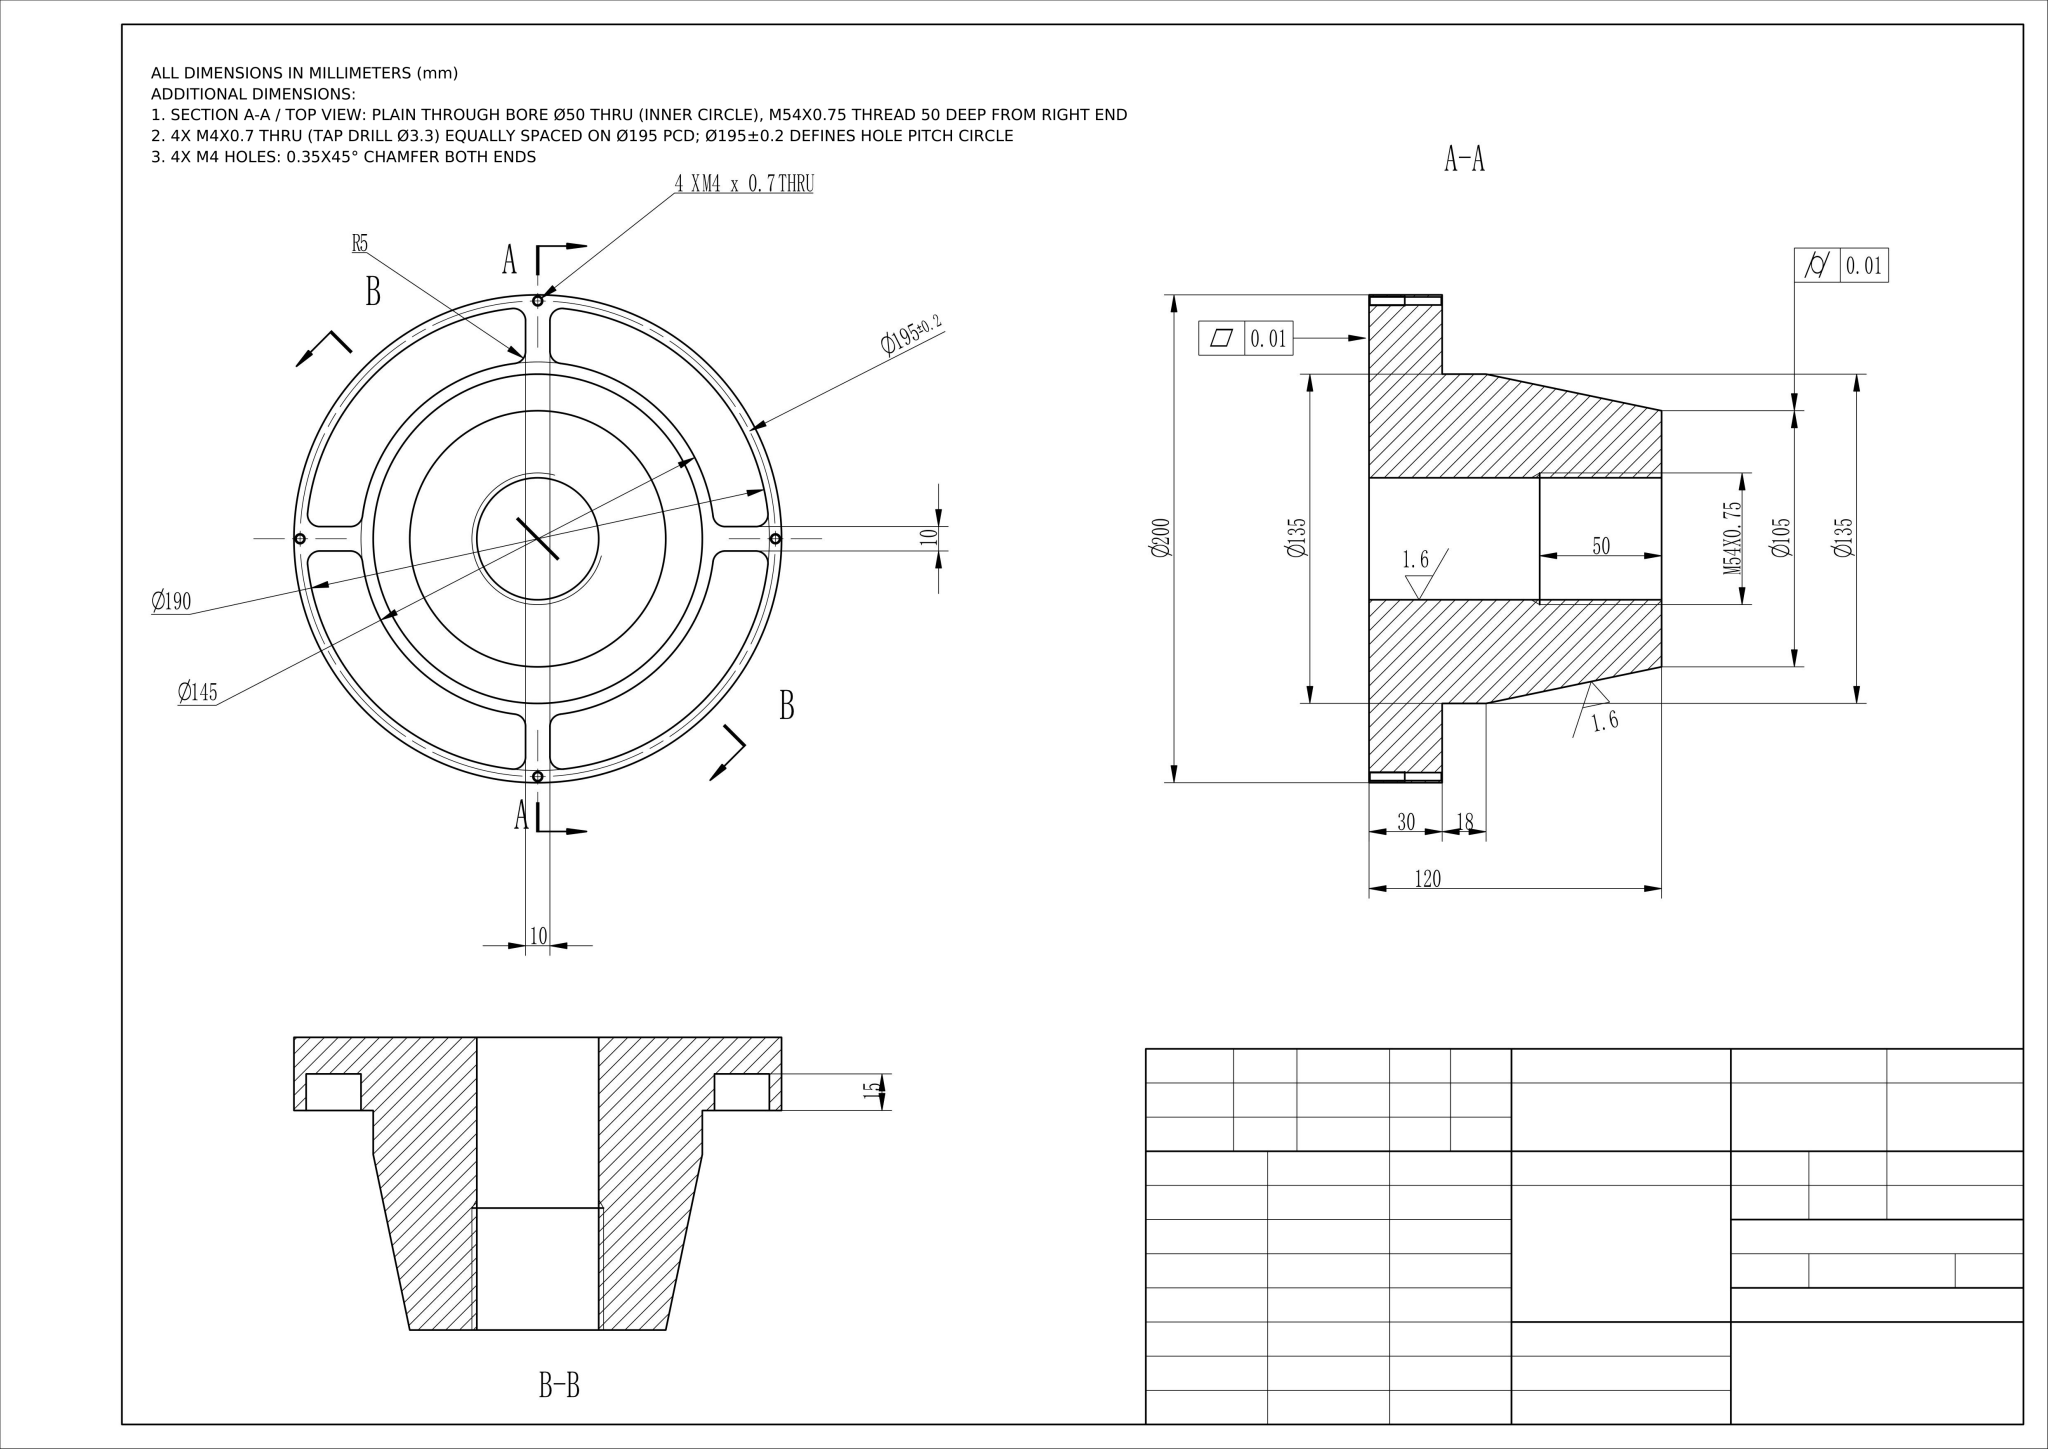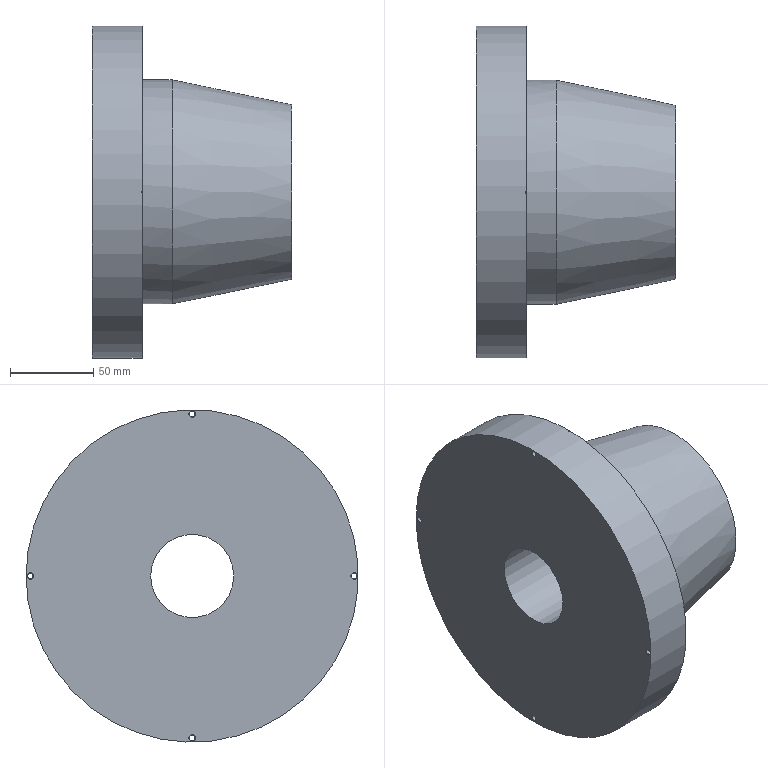Part | NX | mm | 1 solid | 55 faces | box 120 x 200 x 200 mm | volume 1619219 mm3 | cylinder 31 | plane 15 | cone 9 | commonest cylinder face diameters 10 x16 145 x4 190 x4 3.3 x4 200 x1 135 x1 50 x1